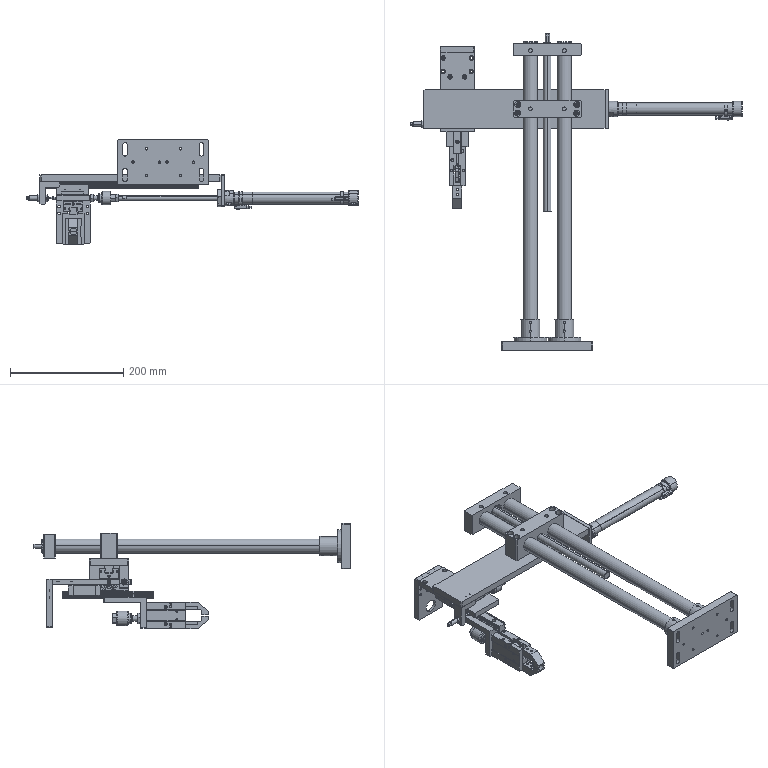Assembly | SolidWorks | mm | 35 component files | 35 solids | 2456 faces | box 586.5 x 559.56 x 185.57 mm | volume 1732685 mm3 | plane 1182 | cylinder 825 | cone 293 | spline 138 | torus 14 | sphere 4 | commonest cylinder face diameters 8 x62 4 x56 0.6 x50 4.2 x48 4.5 x46 3 x42 1.6 x32 6 x29
Bill of materials:
CCDBlankingGripper | 2 | Q235 | Prismatic block with a flat rectangular top, one sloped side face, and a stepped underside. It has a semicircular cutout through the lower end and a filleted inside corner where the step meets the underside.
CCDF-M10X125F | 1 | Q235 | Turned, stepped cylindrical assembly or part. It has a large cylindrical body with a hex section at one end, and a stepped shaft at the other end with a hex nut on it.
CCDJSACA-0806-1_NT | 2 |  | Thin hexagonal nut-like ring with a large central round bore and chamfered corners on both faces.
CCDJSAdjustingScrew01 | 1 |  | Long, slender solid cylindrical rod. One end is stepped down to two smaller-diameter sections.
CCDJSBottomFixingPlate | 1 | 45# | Flat rectangular plate with four elongated slots near the short edges and a pattern of small round through holes.
CCDJSBufferChainBlankingLinearGuide-EGR15R160 | 1 | AISI 304 | Long straight bar with a constant profile. The profile has necked sides with concave grooves and chamfers, and a row of evenly spaced holes runs through the top face.
CCDJSBufferChainBlankingLinearSlider-EGH15CA | 2 |  | Rectangular block with a central channel running through it lengthwise. The channel walls have groove features. The end faces have small round protrusions and a central round recess or hole, plus raised lettering.
CCDJSBufferChainBlanking-Lifting-LinearGuide-EGR15R160 | 1 | AISI 304 | Straight bar with a constant profile like the other rail-like bar but shorter. It has necked sides with concave grooves, and three evenly spaced counterbore-like holes on top.
CCDJSF-M8X125F | 1 |  | Stepped turned assembly or part, similar to the other stepped cylindrical item. It has a large cylindrical body, a hex boss with a central bore at one end, and a stepped shaft with a hex nut at the other.
CCDJSGrippingCylinderAngleAluminum01 | 1 |  | L-shaped bracket. The horizontal leg has a rectangular groove in its top and small holes; the vertical leg has several round through holes of different sizes.
CCDJSHeightAdjustmentBlock01 | 1 | A6061 | Rectangular block with three large cross holes through the long face and several vertical holes through the top face.
CCDJSLiftingCylinderFixingPlate01 | 1 |  | Flat rectangular plate with a pattern of counterbored or plain holes through the face and one hole into a side edge.
CCDJSLiftingCylinderFixingPlate02 | 1 |  | Flat rectangular plate with small chamfered corners. It has a rounded-square through cutout in the upper middle, a large circular through hole in the lower middle, and seven small through holes: three in a row along the top edge and two along each side edge.
CCDJSScrewRodFixingBlock01 | 1 | A6061 | Rectangular block with three large circular through bores side by side through its main face. Two small holes go down from the top face and appear to break into the outer two bores.
CCDJSStopBlock01 | 1 | 45# | Solid L-shaped angle bracket with a filleted inside corner and chamfered outer end corners. The horizontal leg has two through holes in a row, and the vertical leg has one through hole.
CCDJSSupportColumn01 | 2 |  | Plain solid cylindrical rod or pin with flat ends and no visible features.
CCDJSSupportColumnFixingRing01 | 2 | 45# | Flanged cylindrical bushing or hub: a round flange with four evenly spaced through holes, a large central through bore, and a cylindrical hub carrying two radial holes in a row along its length.
CCDJSTransferCylinderFixingPlate01 | 1 | A6061 | Long, thin rectangular bar or plate with small corner chamfers. Four small through holes sit on the main face in two pairs, and three holes are drilled into one end face.
CCDJSTransferCylinderFixingPlate02 | 1 |  | Flat rectangular plate with small chamfered corners. It has three small through holes evenly spaced along one long edge and one large circular through hole near the opposite edge.
Mates:
1. coincident | CCDJSBottomFixingPlate-1 plane at (0, 0, 0) dir (0, 0, 1) | assembly plane at (0, 0, 0) dir (0, 0, 1)
2. coincident | CCDJSBottomFixingPlate-1 plane at (0, 0, 0) dir (0, 1, 0) | assembly plane at (0, 0, 0) dir (0, 1, 0)
3. coincident | CCDJSBottomFixingPlate-1 plane at (0, 0, 0) dir (1, 0, 0) | assembly plane at (0, 0, 0) dir (1, 0, 0)
4. coincident | CCDJSBottomFixingPlate-1 face at (0, 15, 0) dir (0, 1, 0) | CCDJSSupportColumn01-1 face at (30, 15, 0) dir (0, -1, 0)
5. concentric | CCDJSSupportColumnFixingRing01-2 face at (-30, 15, 0) dir (0, -1, 0) r 12.5 | CCDJSSupportColumn01-3 face at (-30, 15, 0) dir (0, 1, 0) r 12.5
6. concentric | CCDJSBottomFixingPlate-1 face at (30, 15, 23.5) dir (0, 1, 0) r 2.1 | CCDJSSupportColumnFixingRing01-3 face at (30, 23, 23.5) dir (0, 1, 0) r 2.75
7. concentric | CCDJSBottomFixingPlate-1 edge at (53.5, 15, 0) dir (0, 1, 0) r 2.1 | CCDJSSupportColumnFixingRing01-3 face at (53.5, 23, 0) dir (0, 1, 0) r 2.75
8. coincident | CCDJSBottomFixingPlate-1 face at (0, 15, 0) dir (0, 1, 0) | CCDJSSupportColumnFixingRing01-3 face at (42.5, 15, 0) dir (0, -1, 0)
9. concentric | CCDJSSupportColumn01-1 face at (30, 15, 0) dir (0, 1, 0) r 12.5 | CCDJSSupportColumnFixingRing01-3 face at (30, 15, 0) dir (0, -1, 0) r 17
10. concentric | CCDJSSupportColumn01-3 face at (-30, 15, 0) dir (0, 1, 0) r 12.5 | CCDJSScrewRodFixingBlock01-2 face at (-30, 541.564, 0) dir (0, -1, 0) r 12.5
11. concentric | CCDJSBottomFixingPlate-1 face at (-53.5, 15, 0) dir (0, 1, 0) r 2.1 | CCDJSSupportColumnFixingRing01-2 face at (-53.5, 23, 0) dir (0, 1, 0) r 2.75
12. concentric | CCDJSBottomFixingPlate-1 edge at (-6.5, 15, 0) dir (0, 1, 0) r 2.1 | CCDJSSupportColumnFixingRing01-2 face at (-6.5, 23, 0) dir (0, 1, 0) r 2.75
13. coincident | CCDJSBottomFixingPlate-1 face at (0, 15, 0) dir (0, 1, 0) | CCDJSSupportColumn01-3 face at (-30, 15, 0) dir (0, -1, 0)
14. coincident | CCDJSBottomFixingPlate-1 face at (0, 15, 0) dir (0, 1, 0) | CCDJSSupportColumnFixingRing01-2 face at (-17.5, 15, 0) dir (0, -1, 0)
15. concentric | CCDJSSupportColumn01-1 face at (30, 15, 0) dir (0, 1, 0) r 12.5 | CCDJSScrewRodFixingBlock01-2 face at (30, 541.564, 0) dir (0, -1, 0) r 12.5
16. concentric | CCDJSScrewRodFixingBlock01-2 face at (0, 560.564, 0) dir (0, -1, 0) r 13 | CCDJSAdjustingScrew01-1 face at (0, 244.564, 0) dir (0, -1, 0) r 7
17. coincident | CCDJSScrewRodFixingBlock01-2 face at (0, 526.564, 0) dir (0, 1, 0) | CCDJSAdjustingScrew01-1 face at (7, 526.564, 0) dir (0, 1, 0)
18. concentric | CCDJSSupportColumn01-3 face at (-30, 15, 0) dir (0, 1, 0) r 12.5 | CCDJSHeightAdjustmentBlock01-1 face at (-30, 446.564, 0) dir (0, -1, 0) r 12.5
19. concentric | CCDJSSupportColumn01-1 face at (30, 15, 0) dir (0, 1, 0) r 12.5 | CCDJSHeightAdjustmentBlock01-1 face at (30, 446.564, 0) dir (0, -1, 0) r 12.5
20. concentric | CCDJSAdjustingScrew01-1 face at (0, 244.564, 0) dir (0, -1, 0) r 7 | CCDJSHeightAdjustmentBlock01-1 face at (0, 411.564, 0) dir (0, -1, 0) r 7
21. coincident | CCDJSHeightAdjustmentBlock01-1 face at (60, 411.564, -22.5) dir (0, 0, -1) | CCDJSTransferCylinderFixingPlate01-1 face at (-218, 461.564, -22.5) dir (0, 0, 1)
22. concentric | CCDJSTransferCylinderFixingPlate01-1 face at (-197.1, 426.564, -34.5) dir (0, 0, -1) r 1.25 | CCDJSBufferChainBlankingLinearGuide-EGH15CA1R160-1/CCDJSBufferChainBlankingLinearGuide-EGR15R160-1 face at (-197.1, 426.564, -47) dir (0, 0, -1) r 1.75
23. coincident | CCDJSTransferCylinderFixingPlate01-1 face at (-218, 461.564, -34.5) dir (0, 0, -1) | CCDJSBufferChainBlankingLinearGuide-EGH15CA1R160-1/CCDJSBufferChainBlankingLinearGuide-EGR15R160-1 face at (62.9, 428.914, -34.5) dir (0, 0, 1)
24. concentric | CCDJSTransferCylinderFixingPlate01-1 edge at (42.9, 426.564, -34.5) dir (0, 0, -1) r 1.25 | CCDJSBufferChainBlankingLinearGuide-EGH15CA1R160-1/CCDJSBufferChainBlankingLinearGuide-EGR15R160-1 face at (42.9, 426.564, -47) dir (0, 0, -1) r 1.75
25. coincident | CCDJSTransferCylinderFixingPlate01-1 face at (102, 461.564, -22.5) dir (1, 0, 0) | CCDJSTransferCylinderFixingPlate02-1 face at (102, 461.564, -22.5) dir (-1, 0, 0)
26. concentric | CCDJSTransferCylinderFixingPlate01-1 face at (102, 451.564, -28.5) dir (1, 0, 0) r 2.1 | CCDJSTransferCylinderFixingPlate02-1 face at (98, 451.564, -28.5) dir (1, 0, 0) r 2.75
27. concentric | CCDJSTransferCylinderFixingPlate01-1 edge at (102, 401.564, -28.5) dir (1, 0, 0) r 2.1 | CCDJSTransferCylinderFixingPlate02-1 face at (98, 401.564, -28.5) dir (1, 0, 0) r 2.75
28. coincident | CCDJSTransferCylinderFixingPlate01-1 face at (-218, 461.564, -34.5) dir (0, 0, -1) | CCDJSStopBlock01-1 face at (-183, 407.564, -34.5) dir (0, 0, 1)
29. concentric | CCDJSTransferCylinderFixingPlate01-1 face at (-189, 399.564, -34.5) dir (0, 0, -1) r 1.65 | CCDJSStopBlock01-1 face at (-189, 399.564, -44.5) dir (0, 0, -1) r 2.25
30. concentric | CCDJSTransferCylinderFixingPlate01-1 face at (-199, 399.564, -34.5) dir (0, 0, -1) r 1.65 | CCDJSStopBlock01-1 face at (-199, 399.564, -44.5) dir (0, 0, -1) r 2.25
31. coincident | CCDJSBufferChainBlankingLinearGuide-EGH15CA1R160-1/CCDJSBufferChainBlankingLinearSlider-EGH15CA-1 face at (-180.4, 410.564, -58.57) dir (0, 0, -1) | CCDJSLiftingCylinderFixingPlate01-1 face at (-159, 456.564, -58.57) dir (0, 0, 1)
32. concentric | CCDJSBufferChainBlankingLinearGuide-EGH15CA1R160-1/CCDJSBufferChainBlankingLinearSlider-EGH15CA-1 face at (-147.5, 439.564, -58.57) dir (0, 0, -1) r 1.65 | CCDJSLiftingCylinderFixingPlate01-1 face at (-147.5, 439.564, -68.57) dir (0, 0, -1) r 2.25
33. concentric | CCDJSBufferChainBlankingLinearGuide-EGH15CA1R160-1/CCDJSBufferChainBlankingLinearSlider-EGH15CA-1 face at (-173.5, 439.564, -58.57) dir (0, 0, -1) r 1.65 | CCDJSLiftingCylinderFixingPlate01-1 face at (-173.5, 439.564, -68.57) dir (0, 0, -1) r 2.25
34. coincident | CCDJSLiftingCylinderFixingPlate01-1 face at (-189, 526.564, -58.57) dir (0, 1, 0) | CCDJSLiftingCylinderFixingPlate02-1 face at (-159, 526.564, -101.07) dir (0, -1, 0)
35. concentric | CCDJSLiftingCylinderFixingPlate01-1 edge at (-144, 526.564, -63.57) dir (0, 1, 0) r 1.65 | CCDJSLiftingCylinderFixingPlate02-1 face at (-144, 536.564, -63.57) dir (0, 1, 0) r 4
36. concentric | CCDJSLiftingCylinderFixingPlate01-1 edge at (-174, 526.564, -63.57) dir (0, 1, 0) r 1.65 | CCDJSLiftingCylinderFixingPlate02-1 face at (-174, 536.564, -63.57) dir (0, 1, 0) r 4
37. concentric | CCDJSLiftingCylinderFixingPlate01-1 face at (-129, 426.564, -63.57) dir (1, 0, 0) r 4 | CCDJSMA20x160SU(0)+(CS1-M-2)-1/CCDJS20UMA160 Rod-1 face at (157, 426.564, -63.57) dir (-1, 0, 0) r 4
38. concentric | CCDJSLiftingCylinderFixingPlate01-1 face at (-129, 426.564, -63.57) dir (1, 0, 0) r 4 | CCDJSF-M8X125F-1 face at (-136, 426.564, -63.57) dir (1, 0, 0) r 4
39. coincident | CCDJSLiftingCylinderFixingPlate01-1 face at (-129, 526.564, -58.57) dir (1, 0, 0) | CCDJSF-M8X125F-1 face at (-129, 430.564, -63.57) dir (-1, 0, 0)
40. coincident | CCDJSMA20x160SU(0)+(CS1-M-2)-1/CCDJS20 MA Nut1-1 face at (-85, 430.475, -59.02) dir (-1, 0, 0) | CCDJSF-M8X125F-1 face at (-85, 430.564, -63.57) dir (1, 0, 0)
41. concentric | CCDJSStopBlock01-1 face at (-218, 399.564, -63.5) dir (-1, 0, 0) r 4 | CCDJSACA0806-1-2/CCDJSACA-0806-1_Body-1 face at (-242.5, 399.564, -63.5) dir (1, 0, 0) r 4
42. coincident | CCDJSStopBlock01-1 face at (-208, 407.564, -74.5) dir (1, 0, 0) | CCDJSACA0806-1-2/CCDJSACA-0806-1_NT-4 face at (-208, 395.61, -64.101) dir (-1, 0, 0)
43. coincident | CCDJSLiftingCylinderFixingPlate01-1 face at (-159, 456.564, -68.57) dir (0, 0, -1) | CCDJSBufferChainBlanking-Z-Axis-LinearGuide-EGH15CA1R160-2/CCDJSBufferChainBlankingLinearSlider-EGH15CA-1 face at (-142.9, 489.964, -68.57) dir (0, 0, 1)
44. concentric | CCDJSLiftingCylinderFixingPlate01-1 face at (-145.9, 483.064, -58.57) dir (0, 0, 1) r 2.25 | CCDJSBufferChainBlanking-Z-Axis-LinearGuide-EGH15CA1R160-2/CCDJSBufferChainBlankingLinearSlider-EGH15CA-1 face at (-145.9, 483.064, -68.57) dir (0, 0, 1) r 1.65
45. concentric | CCDJSLiftingCylinderFixingPlate01-1 face at (-171.9, 483.064, -58.57) dir (0, 0, 1) r 4 | CCDJSBufferChainBlanking-Z-Axis-LinearGuide-EGH15CA1R160-2/CCDJSBufferChainBlankingLinearSlider-EGH15CA-1 face at (-171.9, 483.064, -68.57) dir (0, 0, 1) r 1.65
46. concentric | CCDJSBufferChainBlanking-Z-Axis-LinearGuide-EGH15CA1R160-2/CCDJSBufferChainBlanking-Lifting-LinearGuide-EGR15R160-1 face at (-158.9, 428.464, -80.07) dir (0, 0, 1) r 1.75 | CCDJSGrippingCylinderAngleAluminum01-1 face at (-158.9, 428.464, -100.07) dir (0, 0, -1) r 1.25
47. concentric | CCDJSBufferChainBlanking-Z-Axis-LinearGuide-EGH15CA1R160-2/CCDJSBufferChainBlanking-Lifting-LinearGuide-EGR15R160-1 face at (-158.9, 368.464, -80.07) dir (0, 0, 1) r 3 | CCDJSGrippingCylinderAngleAluminum01-1 face at (-158.9, 368.464, -100.07) dir (0, 0, -1) r 1.25
48. coincident | CCDJSBufferChainBlanking-Z-Axis-LinearGuide-EGH15CA1R160-2/CCDJSBufferChainBlanking-Lifting-LinearGuide-EGR15R160-1 face at (-152.1, 348.464, -92.57) dir (0, 0, -1) | CCDJSGrippingCylinderAngleAluminum01-1 face at (-151.35, 321.364, -92.57) dir (0, 0, 1)
49. concentric | CCDJSHFP20(NC)+(CS1-G-2)-1/CCDJSHFP20_finger(0)-1 edge at (-158.9, 284.664, -106.32) dir (0, 0, -1) r 2 | CCDBlankingGripper-6 face at (-158.9, 284.664, -99.57) dir (0, 0, 1) r 2.1
50. coincident | CCDJSHFP20(NC)+(CS1-G-2)-1/CCDJSHFP20_finger(0)-1 face at (-164.9, 271.064, -106.32) dir (0, 0, 1) | CCDBlankingGripper-6 face at (-166.9, 250.664, -106.32) dir (0, 0, -1)
51. concentric | CCDJSHFP20(NC)+(CS1-G-2)-1/CCDJSHFP20_finger(0)-1 face at (-158.9, 284.664, -132.82) dir (0, 0, -1) r 1.621 | CCDBlankingGripper-8 face at (-158.9, 284.664, -145.57) dir (0, 0, -1) r 2.1
52. coincident | CCDJSHFP20(NC)+(CS1-G-2)-1/CCDJSHFP20_finger(0)-1 face at (-152.9, 306.443, -138.82) dir (0, 0, -1) | CCDBlankingGripper-8 face at (-150.9, 250.664, -138.82) dir (0, 0, 1)
53. coincident | CCDJSGrippingCylinderAngleAluminum01-1 face at (-139.9, 370.364, -145.07) dir (0, 1, 0) | CCDF-M10X125F-1 face at (-165.442, 370.364, -126.158) dir (0, -1, 0)
54. distance | CCDJSTransferCylinderFixingPlate01-1 face at (-58, 461.564, -28.5) dir (0, 1, 0) | CCDJSScrewRodFixingBlock01-2 face at (0, 541.564, 0) dir (0, 1, 0)
55. concentric | CCDJSHeightAdjustmentBlock01-1 face at (52, 434.064, 22.5) dir (0, 0, 1) r 5.5 | CCDJSTransferCylinderFixingPlate01-1 edge at (52, 434.064, -22.5) dir (0, 0, 1) r 2.5
56. concentric | CCDJSHeightAdjustmentBlock01-1 face at (-52, 419.064, 22.5) dir (0, 0, 1) r 5.5 | CCDJSTransferCylinderFixingPlate01-1 face at (-52, 419.064, -22.5) dir (0, 0, 1) r 2.5
57. concentric | CCDJSGrippingCylinderAngleAluminum01-1 edge at (-149.9, 370.364, -138.57) dir (0, 1, 0) r 2.75 | CCDJSHFP20(NC)+(CS1-G-2)-1/CCDJSHFP20_body-1 face at (-149.9, 360.364, -138.57) dir (0, -1, 0) r 2.067
58. concentric | CCDJSGrippingCylinderAngleAluminum01-1 face at (-167.9, 349.364, -106.57) dir (0, 1, 0) r 2.75 | CCDJSHFP20(NC)+(CS1-G-2)-1/CCDJSHFP20_body-1 face at (-167.9, 360.364, -106.57) dir (0, -1, 0) r 2.067
59. coincident | CCDJSGrippingCylinderAngleAluminum01-1 face at (-139.9, 360.364, -90.07) dir (0, -1, 0) | CCDJSHFP20(NC)+(CS1-G-2)-1/CCDJSHFP20_body-1 face at (-158.9, 360.364, -122.57) dir (0, 1, 0)
60. concentric | CCDJSHFP20(NC)+(CS1-G-2)-1/CCDJSHFP20_finger(0)-1 face at (-158.9, 284.664, -132.82) dir (0, 0, -1) r 1.621 | CCDBlankingGripper-8 face at (-158.9, 284.664, -145.57) dir (0, 0, -1) r 2.1
61. concentric | CCDJSACA-0806-1_Body-1 face at (0, 0, 0) dir (0, 1, 0) r 3 | CCDJSACA-0806-1_NT-3 face at (0, 20.5, 0) dir (0, 1, 0) r 3.594
62. distance | CCDJSACA-0806-1_NT-4 face at (3.955, 34.5, -0.6008) dir (0, -1, 0) | CCDJSACA-0806-1_Body-1 face at (0, 52, 0) dir (0, 1, 0)
63. concentric | CCDJSACA-0806-1_Body-1 face at (0, 0, 0) dir (0, 1, 0) r 3.5 | CCDJSACA-0806-1_NT-4 face at (0, 34.5, 0) dir (0, 1, 0) r 3.594
64. distance | CCDJSACA-0806-1_NT-3 face at (4.943, 24.5, -0.751) dir (0, 1, 0) | CCDJSACA-0806-1_NT-4 face at (3.955, 34.5, -0.6008) dir (0, -1, 0)
65. coincident | CCDJSBufferChainBlankingLinearGuide-EGR15R160-1 plane at (0, 0.3, 0) dir (0, 0, 1) | CCDJSBufferChainBlankingLinearGuide-EGH15CA1R160 plane at (0, 0, 0) dir (0, 0, 1)
66. coincident | CCDJSBufferChainBlankingLinearGuide-EGR15R160-1 face at (-2.35, 0, 140) dir (0, -1, 0) | CCDJSBufferChainBlankingLinearGuide-EGH15CA1R160 plane at (0, 0, 0) dir (0, 1, 0)
67. coincident | CCDJSBufferChainBlankingLinearGuide-EGR15R160-1 plane at (0, 0.3, 0) dir (1, 0, 0) | CCDJSBufferChainBlankingLinearGuide-EGH15CA1R160 plane at (0, 0, 0) dir (1, 0, 0)
68. coincident | CCDJSBufferChainBlankingLinearSlider-EGH15CA-1 plane at (0, 24.07, 65.2) dir (1, 0, 0) | CCDJSBufferChainBlankingLinearGuide-EGH15CA1R160 plane at (0, 0, 0) dir (1, 0, 0)
69. distance | CCDJSBufferChainBlankingLinearSlider-EGH15CA-1 face at (0, 24.07, 113.5) dir (0, 0, 1) | CCDJSBufferChainBlankingLinearGuide-EGR15R160-1 face at (7.529, 7.671, 140) dir (0, 0, 1)
70. coincident | CCDJSBufferChainBlankingLinearGuide-EGR15R160-1 face at (-5.831, 12.5, 140) dir (0, 1, 0) | CCDJSBufferChainBlankingLinearSlider-EGH15CA-1 face at (5.831, 12.5, 57.2) dir (0, -1, 0)
71. coincident | CCDJSBufferChainBlanking-Lifting-LinearGuide-EGR15R160-1 plane at (0, 0.3, 0) dir (0, 0, 1) | CCDJSBufferChainBlanking-Z-Axis-LinearGuide-EGH15CA1R160 plane at (0, 0, 0) dir (0, 0, 1)
72. coincident | CCDJSBufferChainBlanking-Lifting-LinearGuide-EGR15R160-1 face at (-2.35, 0, 80) dir (0, -1, 0) | CCDJSBufferChainBlanking-Z-Axis-LinearGuide-EGH15CA1R160 plane at (0, 0, 0) dir (0, 1, 0)
73. coincident | CCDJSBufferChainBlanking-Lifting-LinearGuide-EGR15R160-1 plane at (0, 0.3, 0) dir (1, 0, 0) | CCDJSBufferChainBlanking-Z-Axis-LinearGuide-EGH15CA1R160 plane at (0, 0, 0) dir (1, 0, 0)
74. coincident | CCDJSBufferChainBlankingLinearSlider-EGH15CA-1 plane at (0, 24, -61.5) dir (1, 0, 0) | CCDJSBufferChainBlanking-Z-Axis-LinearGuide-EGH15CA1R160 plane at (0, 0, 0) dir (1, 0, 0)
75. distance | CCDJSBufferChainBlankingLinearSlider-EGH15CA-1 face at (16, 24, -61.5) dir (0, 1, 0) | CCDJSBufferChainBlanking-Lifting-LinearGuide-EGR15R160-1 face at (6.8, 0, 80) dir (0, -1, 0)
76. distance | CCDJSBufferChainBlankingLinearSlider-EGH15CA-1 face at (0, 24, -70) dir (0, 0, -1) | CCDJSBufferChainBlanking-Lifting-LinearGuide-EGR15R160-1 face at (7.529, 7.671, -80) dir (0, 0, -1)
77. distance | CCDJSHFP20_body-1 plane at (0, 0, 0) dir (-1, 0, 0) | CCDJSHFP20(0-G-2)_dummy-1 plane at (0, 0, 0) dir (1, 0, 0)
78. coincident | CCDJSHFP20(0-G-2)_dummy-1 axis at (80.9, 0, 0) dir (-1, 0, 0) | CCDJSHFP20_body-1 axis at (-80.9, 0, 0) dir (1, 0, 0)
79. angle | CCDJSHFP20_body-1 plane at (0, 0, 0) dir (0, 0, 1) | CCDJSHFP20(0-G-2)_dummy-1 plane at (0, 0, 0) dir (0, 0, -1)
80. distance | CCDJSHFP20_finger(0)-1 plane at (0, 0, 0) dir (1, 0, 0) | CCDJSHFP20_body-1 plane at (0, 0, 0) dir (-1, 0, 0)
81. coincident | CCDJSHFP20_body-1 axis at (-80.9, 0, 0) dir (1, 0, 0) | CCDJSHFP20_finger(0)-1 axis at (80.9, 0, 0) dir (-1, 0, 0)
82. angle | CCDJSHFP20_finger(0)-1 plane at (0, 0, 0) dir (0, 0, 1) | CCDJSHFP20_body-1 plane at (0, 0, 0) dir (0, 0, 1)
83. distance | CCDJSCS1-G()-1 plane at (43.5, -12, 0) dir (1, 0, 0) | CCDJSHFP20_body-1 plane at (69, 0, 0) dir (1, 0, 0)
84. coincident | CCDJSHFP20_body-1 axis at (80.9, -12, 0) dir (-1, 0, 0) | CCDJSCS1-G()-1 axis at (124.4, -12, 0) dir (-1, 0, 0)
85. angle | CCDJSCS1-G()-1 plane at (43.5, -12, 0) dir (0, 0, 1) | CCDJSHFP20_body-1 plane at (0, 0, 0) dir (0, 0, 1)
86. distance | CCDJSCS1-G()-2 plane at (35.4, 12, 0) dir (1, 0, 0) | CCDJSHFP20_body-1 plane at (69, 0, 0) dir (1, 0, 0)
87. coincident | CCDJSHFP20_body-1 axis at (80.9, 12, 0) dir (-1, 0, 0) | CCDJSCS1-G()-2 axis at (116.3, 12, 0) dir (-1, 0, 0)
88. angle | CCDJSCS1-G()-2 plane at (35.4, 12, 0) dir (0, 0, -1) | CCDJSHFP20_body-1 plane at (0, 0, 0) dir (0, 0, 1)
89. coincident | CCDJS20MAU160 Body-1 axis at (-108.9, 0, 0) dir (1, 0, 0) | CCDJS20UMA160 Rod-1 axis at (-296.9, 0, 0) dir (1, 0, 0)
90. angle | CCDJS20UMA160 Rod-1 plane at (-216, 0, 0) dir (0, 0, -1) | CCDJS20MAU160 Body-1 plane at (-28, 0, 0) dir (0, 0, -1)
91. coincident | CCDJS20MAU160 Body-1 axis at (-108.9, 0, 0) dir (1, 0, 0) | CCDJS20 MA Nut-1 axis at (-108.9, 0, 0) dir (1, 0, 0)
92. angle | CCDJS20 MA Nut-1 plane at (-28, 0, 0) dir (0, 0, -1) | CCDJS20MAU160 Body-1 plane at (-28, 0, 0) dir (0, 0, -1)
93. coincident | CCDJS20MAU160 Body-1 axis at (-108.9, 0, 0) dir (1, 0, 0) | CCDJS20 MA Nut1-1 axis at (-125.1, 0, 0) dir (-1, 0, 0)
94. angle | CCDJS20 MA Nut1-1 plane at (-206, 0, 0) dir (0, 0, -1) | CCDJS20MAU160 Body-1 plane at (-28, 0, 0) dir (0, 0, -1)
95. distance | CCDJSCS1-M-S20-1 plane at (1, 0, 0) dir (1, 0, 0) | CCDJS20MAU160 Body-1 plane at (1, 0, 0) dir (-1, 0, 0)
96. coincident | CCDJS20MAU160 Body-1 axis at (-108.9, 0, 0) dir (1, 0, 0) | CCDJSCS1-M-S20-1 axis at (81.9, 0, 0) dir (-1, 0, 0)
97. angle | CCDJSCS1-M-S20-1 plane at (1, 0, 0) dir (0, 0.7071, -0.7071) | CCDJS20MAU160 Body-1 plane at (-28, 0, 0) dir (0, 0, -1)
98. distance | CCDJSCS1-M-S20-2 plane at (203, 0, 0) dir (-1, 0, 0) | CCDJS20MAU160 Body-1 plane at (203, 0, 0) dir (1, 0, 0)
99. coincident | CCDJS20MAU160 Body-1 axis at (52.9, 0, 0) dir (-1, 0, 0) | CCDJSCS1-M-S20-2 axis at (122.1, 0, 0) dir (1, 0, 0)
100. angle | CCDJSCS1-M-S20-2 plane at (203, 0, 0) dir (0, 0.7071, 0.7071) | CCDJS20MAU160 Body-1 plane at (-28, 0, 0) dir (0, 0, -1)
101. distance | CCDJS20UMA160 Rod-1 face at (-216, 0, 0) dir (-1, 0, 0) | CCDJS20MAU160 Body-1 face at (-16, 11, 0) dir (-1, 0, 0)
102. distance | CCDJS20UMA160 Rod-1 face at (-216, 0, 0) dir (-1, 0, 0) | CCDJS20 MA Nut1-1 face at (-209, -6, 0) dir (-1, 0, 0)
103. distance | CCDJS20MAU160 Body-1 face at (-16, 11, 0) dir (-1, 0, 0) | CCDJS20 MA Nut-1 face at (-21, 14.2, 0) dir (1, 0, 0)